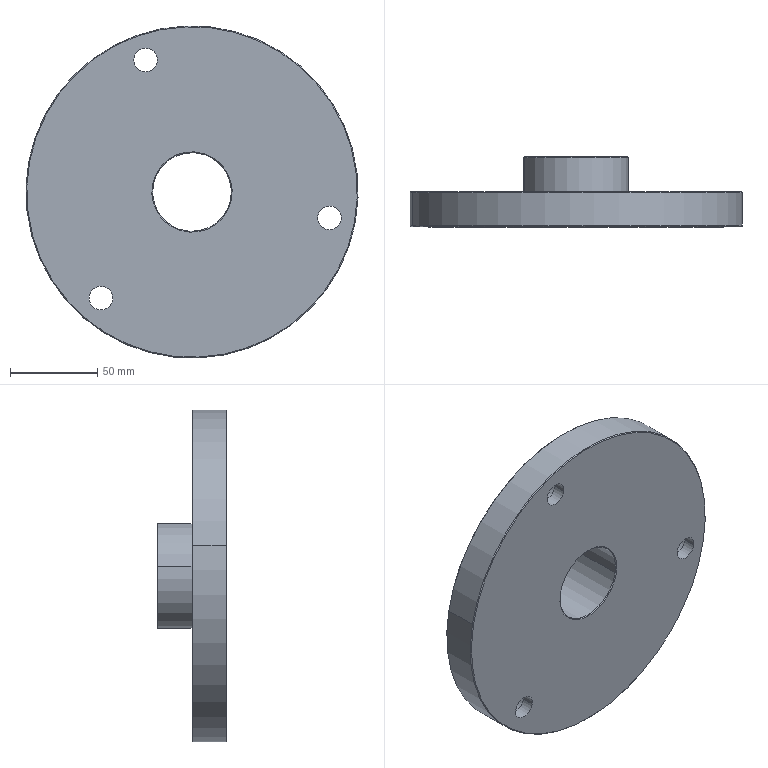Component | SolidWorks | 002AS-20130718-1_009A-20130717-1 | 1 solid | 34 faces | box 190 x 40 x 190 mm | volume 544523 mm3 | cylinder 18 | cone 10 | plane 6 | commonest cylinder face diameters 20 x6 13.5 x6 60 x2 45 x2 190 x2
STEP:
#1=COLOUR_RGB('',0.7922,0.8196,0.9333);
#2=FILL_AREA_STYLE_COLOUR('',#1);
#3=FILL_AREA_STYLE('',(#2));
#4=SURFACE_STYLE_FILL_AREA(#3);
#5=SURFACE_SIDE_STYLE('',(#4));
#6=SURFACE_STYLE_USAGE(.BOTH.,#5);
#7=PRESENTATION_STYLE_ASSIGNMENT((#6));
#8=CARTESIAN_POINT('',(-10.319,22.763,3.707));
#9=VERTEX_POINT('',#8);
#10=CARTESIAN_POINT('',(-8.578,22.763,3.38));
#11=VERTEX_POINT('',#10);
#12=CARTESIAN_POINT('',(-9.449,22.763,3.543));
#13=DIRECTION('',(-0.,-1.,0.));
#14=DIRECTION('',(-0.9828,0.,0.1846));
#15=AXIS2_PLACEMENT_3D('',#12,#13,#14);
#16=CIRCLE('',#15,0.8858);
#17=EDGE_CURVE('',#9,#11,#16,.T.);
#18=ORIENTED_EDGE('',*,*,#17,.F.);
#19=CARTESIAN_POINT('',(-10.339,22.743,3.71));
#20=VERTEX_POINT('',#19);
#21=CARTESIAN_POINT('',(-10.339,22.743,3.71));
#22=DIRECTION('',(-0.695,-0.7071,0.1305));
#23=VECTOR('',#22,39.37);
#24=LINE('',#21,#23);
#25=EDGE_CURVE('',#9,#20,#24,.T.);
#26=ORIENTED_EDGE('',*,*,#25,.T.);
#27=CARTESIAN_POINT('',(-8.559,22.743,3.376));
#28=VERTEX_POINT('',#27);
#29=CARTESIAN_POINT('',(-9.449,22.743,3.543));
#30=DIRECTION('',(0.,1.,-0.));
#31=DIRECTION('',(-0.9828,0.,0.1846));
#32=AXIS2_PLACEMENT_3D('',#29,#30,#31);
#33=CIRCLE('',#32,0.9055);
#34=EDGE_CURVE('',#28,#20,#33,.T.);
#35=ORIENTED_EDGE('',*,*,#34,.F.);
#36=CARTESIAN_POINT('',(-8.559,22.743,3.376));
#37=DIRECTION('',(0.695,-0.7071,-0.1305));
#38=VECTOR('',#37,39.37);
#39=LINE('',#36,#38);
#40=EDGE_CURVE('',#11,#28,#39,.T.);
#41=ORIENTED_EDGE('',*,*,#40,.F.);
#42=EDGE_LOOP('',(#18,#26,#35,#41));
#43=FACE_OUTER_BOUND('',#42,.T.);
#44=CARTESIAN_POINT('',(-9.449,22.743,3.543));
#45=DIRECTION('',(-0.,-1.,0.));
#46=DIRECTION('',(0.9828,0.,-0.1846));
#47=AXIS2_PLACEMENT_3D('',#44,#45,#46);
#48=CONICAL_SURFACE('',#47,0.9055,0.7854);
#49=ADVANCED_FACE('',(#43),#48,.F.);
#50=CARTESIAN_POINT('',(-10.59,24.318,3.758));
#51=VERTEX_POINT('',#50);
#52=CARTESIAN_POINT('',(-8.307,24.318,3.329));
#53=VERTEX_POINT('',#52);
#54=CARTESIAN_POINT('',(-9.449,24.318,3.543));
#55=DIRECTION('',(0.,1.,-0.));
#56=DIRECTION('',(-0.9828,0.,0.1846));
#57=AXIS2_PLACEMENT_3D('',#54,#55,#56);
#58=CIRCLE('',#57,1.161);
#59=EDGE_CURVE('',#51,#53,#58,.T.);
#60=ORIENTED_EDGE('',*,*,#59,.F.);
#61=CARTESIAN_POINT('',(-10.61,24.298,3.761));
#62=VERTEX_POINT('',#61);
#63=CARTESIAN_POINT('',(-10.59,24.318,3.758));
#64=DIRECTION('',(-0.695,-0.7071,0.1305));
#65=VECTOR('',#64,39.37);
#66=LINE('',#63,#65);
#67=EDGE_CURVE('',#51,#62,#66,.T.);
#68=ORIENTED_EDGE('',*,*,#67,.T.);
#69=CARTESIAN_POINT('',(-8.288,24.298,3.325));
#70=VERTEX_POINT('',#69);
#71=CARTESIAN_POINT('',(-9.449,24.298,3.543));
#72=DIRECTION('',(-0.,-1.,0.));
#73=DIRECTION('',(-0.9828,0.,0.1846));
#74=AXIS2_PLACEMENT_3D('',#71,#72,#73);
#75=CIRCLE('',#74,1.181);
#76=EDGE_CURVE('',#70,#62,#75,.T.);
#77=ORIENTED_EDGE('',*,*,#76,.F.);
#78=CARTESIAN_POINT('',(-8.307,24.318,3.329));
#79=DIRECTION('',(0.695,-0.7071,-0.1305));
#80=VECTOR('',#79,39.37);
#81=LINE('',#78,#80);
#82=EDGE_CURVE('',#53,#70,#81,.T.);
#83=ORIENTED_EDGE('',*,*,#82,.F.);
#84=EDGE_LOOP('',(#60,#68,#77,#83));
#85=FACE_OUTER_BOUND('',#84,.T.);
#86=CARTESIAN_POINT('',(-9.449,24.318,3.543));
#87=DIRECTION('',(-0.,-1.,0.));
#88=DIRECTION('',(0.9828,0.,-0.1846));
#89=AXIS2_PLACEMENT_3D('',#86,#87,#88);
#90=CONICAL_SURFACE('',#89,1.161,0.7854);
#91=ADVANCED_FACE('',(#85),#90,.T.);
#92=CARTESIAN_POINT('',(-8.578,24.298,3.38));
#93=VERTEX_POINT('',#92);
#94=CARTESIAN_POINT('',(-10.319,24.298,3.707));
#95=VERTEX_POINT('',#94);
#96=CARTESIAN_POINT('',(-9.449,24.298,3.543));
#97=DIRECTION('',(0.,1.,-0.));
#98=DIRECTION('',(-0.9828,0.,0.1846));
#99=AXIS2_PLACEMENT_3D('',#96,#97,#98);
#100=CIRCLE('',#99,0.8858);
#101=EDGE_CURVE('',#93,#95,#100,.T.);
#102=ORIENTED_EDGE('',*,*,#101,.F.);
#103=CARTESIAN_POINT('',(-8.559,24.318,3.376));
#104=VERTEX_POINT('',#103);
#105=CARTESIAN_POINT('',(-8.578,24.298,3.38));
#106=DIRECTION('',(0.695,0.7071,-0.1305));
#107=VECTOR('',#106,39.37);
#108=LINE('',#105,#107);
#109=EDGE_CURVE('',#93,#104,#108,.T.);
#110=ORIENTED_EDGE('',*,*,#109,.T.);
#111=CARTESIAN_POINT('',(-10.339,24.318,3.71));
#112=VERTEX_POINT('',#111);
#113=CARTESIAN_POINT('',(-9.449,24.318,3.543));
#114=DIRECTION('',(-0.,-1.,0.));
#115=DIRECTION('',(-0.9828,0.,0.1846));
#116=AXIS2_PLACEMENT_3D('',#113,#114,#115);
#117=CIRCLE('',#116,0.9055);
#118=EDGE_CURVE('',#112,#104,#117,.T.);
#119=ORIENTED_EDGE('',*,*,#118,.F.);
#120=CARTESIAN_POINT('',(-10.319,24.298,3.707));
#121=DIRECTION('',(-0.695,0.7071,0.1305));
#122=VECTOR('',#121,39.37);
#123=LINE('',#120,#122);
#124=EDGE_CURVE('',#95,#112,#123,.T.);
#125=ORIENTED_EDGE('',*,*,#124,.F.);
#126=EDGE_LOOP('',(#102,#110,#119,#125));
#127=FACE_OUTER_BOUND('',#126,.T.);
#128=CARTESIAN_POINT('',(-9.449,24.298,3.543));
#129=DIRECTION('',(0.,1.,-0.));
#130=DIRECTION('',(-0.9828,0.,0.1846));
#131=AXIS2_PLACEMENT_3D('',#128,#129,#130);
#132=CONICAL_SURFACE('',#131,0.8858,0.7854);
#133=ADVANCED_FACE('',(#127),#132,.F.);
#134=CARTESIAN_POINT('',(-11.113,23.019,1.081));
#135=VERTEX_POINT('',#134);
#136=CARTESIAN_POINT('',(-11.887,23.019,1.226));
#137=VERTEX_POINT('',#136);
#138=CARTESIAN_POINT('',(-11.5,23.019,1.153));
#139=DIRECTION('',(0.,1.,-0.));
#140=DIRECTION('',(-0.9828,0.,0.1846));
#141=AXIS2_PLACEMENT_3D('',#138,#139,#140);
#142=CIRCLE('',#141,0.3937);
#143=EDGE_CURVE('',#135,#137,#142,.T.);
#144=ORIENTED_EDGE('',*,*,#143,.F.);
#145=CARTESIAN_POINT('',(-11.113,23.531,1.081));
#146=VERTEX_POINT('',#145);
#147=CARTESIAN_POINT('',(-11.113,23.531,1.081));
#148=DIRECTION('',(0.,1.,-0.));
#149=VECTOR('',#148,39.37);
#150=LINE('',#147,#149);
#151=EDGE_CURVE('',#135,#146,#150,.T.);
#152=ORIENTED_EDGE('',*,*,#151,.T.);
#153=CARTESIAN_POINT('',(-11.887,23.531,1.226));
#154=VERTEX_POINT('',#153);
#155=CARTESIAN_POINT('',(-11.5,23.531,1.153));
#156=DIRECTION('',(0.,1.,-0.));
#157=DIRECTION('',(-0.9828,0.,0.1846));
#158=AXIS2_PLACEMENT_3D('',#155,#156,#157);
#159=CIRCLE('',#158,0.3937);
#160=EDGE_CURVE('',#146,#154,#159,.T.);
#161=ORIENTED_EDGE('',*,*,#160,.T.);
#162=CARTESIAN_POINT('',(-11.887,23.531,1.226));
#163=DIRECTION('',(0.,1.,-0.));
#164=VECTOR('',#163,39.37);
#165=LINE('',#162,#164);
#166=EDGE_CURVE('',#137,#154,#165,.T.);
#167=ORIENTED_EDGE('',*,*,#166,.F.);
#168=EDGE_LOOP('',(#144,#152,#161,#167));
#169=FACE_OUTER_BOUND('',#168,.T.);
#170=CARTESIAN_POINT('',(-11.5,23.531,1.153));
#171=DIRECTION('',(0.,1.,-0.));
#172=DIRECTION('',(-0.9828,0.,0.1846));
#173=AXIS2_PLACEMENT_3D('',#170,#171,#172);
#174=CYLINDRICAL_SURFACE('',#173,0.3937);
#175=ADVANCED_FACE('',(#169),#174,.F.);
#176=CARTESIAN_POINT('',(-11.239,22.743,1.104));
#177=VERTEX_POINT('',#176);
#178=CARTESIAN_POINT('',(-11.761,22.743,1.202));
#179=VERTEX_POINT('',#178);
#180=CARTESIAN_POINT('',(-11.5,22.743,1.153));
#181=DIRECTION('',(0.,1.,-0.));
#182=DIRECTION('',(-0.9828,0.,0.1846));
#183=AXIS2_PLACEMENT_3D('',#180,#181,#182);
#184=CIRCLE('',#183,0.2657);
#185=EDGE_CURVE('',#177,#179,#184,.T.);
#186=ORIENTED_EDGE('',*,*,#185,.F.);
#187=CARTESIAN_POINT('',(-11.239,23.019,1.104));
#188=VERTEX_POINT('',#187);
#189=CARTESIAN_POINT('',(-11.239,23.531,1.104));
#190=DIRECTION('',(0.,1.,-0.));
#191=VECTOR('',#190,39.37);
#192=LINE('',#189,#191);
#193=EDGE_CURVE('',#177,#188,#192,.T.);
#194=ORIENTED_EDGE('',*,*,#193,.T.);
#195=CARTESIAN_POINT('',(-11.761,23.019,1.202));
#196=VERTEX_POINT('',#195);
#197=CARTESIAN_POINT('',(-11.5,23.019,1.153));
#198=DIRECTION('',(0.,1.,-0.));
#199=DIRECTION('',(-0.9828,0.,0.1846));
#200=AXIS2_PLACEMENT_3D('',#197,#198,#199);
#201=CIRCLE('',#200,0.2657);
#202=EDGE_CURVE('',#188,#196,#201,.T.);
#203=ORIENTED_EDGE('',*,*,#202,.T.);
#204=CARTESIAN_POINT('',(-11.761,23.531,1.202));
#205=DIRECTION('',(0.,1.,-0.));
#206=VECTOR('',#205,39.37);
#207=LINE('',#204,#206);
#208=EDGE_CURVE('',#179,#196,#207,.T.);
#209=ORIENTED_EDGE('',*,*,#208,.F.);
#210=EDGE_LOOP('',(#186,#194,#203,#209));
#211=FACE_OUTER_BOUND('',#210,.T.);
#212=CARTESIAN_POINT('',(-11.5,23.531,1.153));
#213=DIRECTION('',(0.,1.,-0.));
#214=DIRECTION('',(-0.9828,0.,0.1846));
#215=AXIS2_PLACEMENT_3D('',#212,#213,#214);
#216=CYLINDRICAL_SURFACE('',#215,0.2657);
#217=ADVANCED_FACE('',(#211),#216,.F.);
#218=CARTESIAN_POINT('',(-10.106,23.019,6.442));
#219=VERTEX_POINT('',#218);
#220=CARTESIAN_POINT('',(-10.88,23.019,6.587));
#221=VERTEX_POINT('',#220);
#222=CARTESIAN_POINT('',(-10.493,23.019,6.515));
#223=DIRECTION('',(0.,1.,-0.));
#224=DIRECTION('',(-0.9828,0.,0.1846));
#225=AXIS2_PLACEMENT_3D('',#222,#223,#224);
#226=CIRCLE('',#225,0.3937);
#227=EDGE_CURVE('',#219,#221,#226,.T.);
#228=ORIENTED_EDGE('',*,*,#227,.F.);
#229=CARTESIAN_POINT('',(-10.106,23.531,6.442));
#230=VERTEX_POINT('',#229);
#231=CARTESIAN_POINT('',(-10.106,23.531,6.442));
#232=DIRECTION('',(0.,1.,-0.));
#233=VECTOR('',#232,39.37);
#234=LINE('',#231,#233);
#235=EDGE_CURVE('',#219,#230,#234,.T.);
#236=ORIENTED_EDGE('',*,*,#235,.T.);
#237=CARTESIAN_POINT('',(-10.88,23.531,6.587));
#238=VERTEX_POINT('',#237);
#239=CARTESIAN_POINT('',(-10.493,23.531,6.515));
#240=DIRECTION('',(0.,1.,-0.));
#241=DIRECTION('',(-0.9828,0.,0.1846));
#242=AXIS2_PLACEMENT_3D('',#239,#240,#241);
#243=CIRCLE('',#242,0.3937);
#244=EDGE_CURVE('',#230,#238,#243,.T.);
#245=ORIENTED_EDGE('',*,*,#244,.T.);
#246=CARTESIAN_POINT('',(-10.88,23.531,6.587));
#247=DIRECTION('',(0.,1.,-0.));
#248=VECTOR('',#247,39.37);
#249=LINE('',#246,#248);
#250=EDGE_CURVE('',#221,#238,#249,.T.);
#251=ORIENTED_EDGE('',*,*,#250,.F.);
#252=EDGE_LOOP('',(#228,#236,#245,#251));
#253=FACE_OUTER_BOUND('',#252,.T.);
#254=CARTESIAN_POINT('',(-10.493,23.531,6.515));
#255=DIRECTION('',(0.,1.,-0.));
#256=DIRECTION('',(-0.9828,0.,0.1846));
#257=AXIS2_PLACEMENT_3D('',#254,#255,#256);
#258=CYLINDRICAL_SURFACE('',#257,0.3937);
#259=ADVANCED_FACE('',(#253),#258,.F.);
#260=CARTESIAN_POINT('',(-10.232,22.743,6.466));
#261=VERTEX_POINT('',#260);
#262=CARTESIAN_POINT('',(-10.754,22.743,6.564));
#263=VERTEX_POINT('',#262);
#264=CARTESIAN_POINT('',(-10.493,22.743,6.515));
#265=DIRECTION('',(0.,1.,-0.));
#266=DIRECTION('',(-0.9828,0.,0.1846));
#267=AXIS2_PLACEMENT_3D('',#264,#265,#266);
#268=CIRCLE('',#267,0.2657);
#269=EDGE_CURVE('',#261,#263,#268,.T.);
#270=ORIENTED_EDGE('',*,*,#269,.F.);
#271=CARTESIAN_POINT('',(-10.232,23.019,6.466));
#272=VERTEX_POINT('',#271);
#273=CARTESIAN_POINT('',(-10.232,23.531,6.466));
#274=DIRECTION('',(0.,1.,-0.));
#275=VECTOR('',#274,39.37);
#276=LINE('',#273,#275);
#277=EDGE_CURVE('',#261,#272,#276,.T.);
#278=ORIENTED_EDGE('',*,*,#277,.T.);
#279=CARTESIAN_POINT('',(-10.754,23.019,6.564));
#280=VERTEX_POINT('',#279);
#281=CARTESIAN_POINT('',(-10.493,23.019,6.515));
#282=DIRECTION('',(0.,1.,-0.));
#283=DIRECTION('',(-0.9828,0.,0.1846));
#284=AXIS2_PLACEMENT_3D('',#281,#282,#283);
#285=CIRCLE('',#284,0.2657);
#286=EDGE_CURVE('',#272,#280,#285,.T.);
#287=ORIENTED_EDGE('',*,*,#286,.T.);
#288=CARTESIAN_POINT('',(-10.754,23.531,6.564));
#289=DIRECTION('',(0.,1.,-0.));
#290=VECTOR('',#289,39.37);
#291=LINE('',#288,#290);
#292=EDGE_CURVE('',#263,#280,#291,.T.);
#293=ORIENTED_EDGE('',*,*,#292,.F.);
#294=EDGE_LOOP('',(#270,#278,#287,#293));
#295=FACE_OUTER_BOUND('',#294,.T.);
#296=CARTESIAN_POINT('',(-10.493,23.531,6.515));
#297=DIRECTION('',(0.,1.,-0.));
#298=DIRECTION('',(-0.9828,0.,0.1846));
#299=AXIS2_PLACEMENT_3D('',#296,#297,#298);
#300=CYLINDRICAL_SURFACE('',#299,0.2657);
#301=ADVANCED_FACE('',(#295),#300,.F.);
#302=CARTESIAN_POINT('',(-13.105,23.531,4.23));
#303=VERTEX_POINT('',#302);
#304=CARTESIAN_POINT('',(-5.792,23.531,2.857));
#305=VERTEX_POINT('',#304);
#306=CARTESIAN_POINT('',(-9.449,23.531,3.543));
#307=DIRECTION('',(0.,1.,-0.));
#308=DIRECTION('',(-0.9828,0.,0.1846));
#309=AXIS2_PLACEMENT_3D('',#306,#307,#308);
#310=CIRCLE('',#309,3.72);
#311=EDGE_CURVE('',#303,#305,#310,.T.);
#312=ORIENTED_EDGE('',*,*,#311,.F.);
#313=CARTESIAN_POINT('',(-13.125,23.511,4.234));
#314=VERTEX_POINT('',#313);
#315=CARTESIAN_POINT('',(-13.105,23.531,4.23));
#316=DIRECTION('',(-0.695,-0.7071,0.1305));
#317=VECTOR('',#316,39.37);
#318=LINE('',#315,#317);
#319=EDGE_CURVE('',#303,#314,#318,.T.);
#320=ORIENTED_EDGE('',*,*,#319,.T.);
#321=CARTESIAN_POINT('',(-5.773,23.511,2.853));
#322=VERTEX_POINT('',#321);
#323=CARTESIAN_POINT('',(-9.449,23.511,3.543));
#324=DIRECTION('',(-0.,-1.,0.));
#325=DIRECTION('',(-0.9828,0.,0.1846));
#326=AXIS2_PLACEMENT_3D('',#323,#324,#325);
#327=CIRCLE('',#326,3.74);
#328=EDGE_CURVE('',#322,#314,#327,.T.);
#329=ORIENTED_EDGE('',*,*,#328,.F.);
#330=CARTESIAN_POINT('',(-5.792,23.531,2.857));
#331=DIRECTION('',(0.695,-0.7071,-0.1305));
#332=VECTOR('',#331,39.37);
#333=LINE('',#330,#332);
#334=EDGE_CURVE('',#305,#322,#333,.T.);
#335=ORIENTED_EDGE('',*,*,#334,.F.);
#336=EDGE_LOOP('',(#312,#320,#329,#335));
#337=FACE_OUTER_BOUND('',#336,.T.);
#338=CARTESIAN_POINT('',(-9.449,23.531,3.543));
#339=DIRECTION('',(-0.,-1.,0.));
#340=DIRECTION('',(0.9828,0.,-0.1846));
#341=AXIS2_PLACEMENT_3D('',#338,#339,#340);
#342=CONICAL_SURFACE('',#341,3.72,0.7854);
#343=ADVANCED_FACE('',(#337),#342,.T.);
#344=CARTESIAN_POINT('',(-5.792,22.743,2.857));
#345=VERTEX_POINT('',#344);
#346=CARTESIAN_POINT('',(-13.105,22.743,4.23));
#347=VERTEX_POINT('',#346);
#348=CARTESIAN_POINT('',(-9.449,22.743,3.543));
#349=DIRECTION('',(-0.,-1.,0.));
#350=DIRECTION('',(-0.9828,0.,0.1846));
#351=AXIS2_PLACEMENT_3D('',#348,#349,#350);
#352=CIRCLE('',#351,3.72);
#353=EDGE_CURVE('',#345,#347,#352,.T.);
#354=ORIENTED_EDGE('',*,*,#353,.F.);
#355=CARTESIAN_POINT('',(-5.773,22.763,2.853));
#356=VERTEX_POINT('',#355);
#357=CARTESIAN_POINT('',(-5.773,22.763,2.853));
#358=DIRECTION('',(0.695,0.7071,-0.1305));
#359=VECTOR('',#358,39.37);
#360=LINE('',#357,#359);
#361=EDGE_CURVE('',#345,#356,#360,.T.);
#362=ORIENTED_EDGE('',*,*,#361,.T.);
#363=CARTESIAN_POINT('',(-13.125,22.763,4.234));
#364=VERTEX_POINT('',#363);
#365=CARTESIAN_POINT('',(-9.449,22.763,3.543));
#366=DIRECTION('',(0.,1.,-0.));
#367=DIRECTION('',(-0.9828,0.,0.1846));
#368=AXIS2_PLACEMENT_3D('',#365,#366,#367);
#369=CIRCLE('',#368,3.74);
#370=EDGE_CURVE('',#364,#356,#369,.T.);
#371=ORIENTED_EDGE('',*,*,#370,.F.);
#372=CARTESIAN_POINT('',(-13.125,22.763,4.234));
#373=DIRECTION('',(-0.695,0.7071,0.1305));
#374=VECTOR('',#373,39.37);
#375=LINE('',#372,#374);
#376=EDGE_CURVE('',#347,#364,#375,.T.);
#377=ORIENTED_EDGE('',*,*,#376,.F.);
#378=EDGE_LOOP('',(#354,#362,#371,#377));
#379=FACE_OUTER_BOUND('',#378,.T.);
#380=CARTESIAN_POINT('',(-9.449,22.763,3.543));
#381=DIRECTION('',(0.,1.,-0.));
#382=DIRECTION('',(-0.9828,0.,0.1846));
#383=AXIS2_PLACEMENT_3D('',#380,#381,#382);
#384=CONICAL_SURFACE('',#383,3.74,0.7854);
#385=ADVANCED_FACE('',(#379),#384,.T.);
#386=CARTESIAN_POINT('',(-5.966,23.019,2.889));
#387=VERTEX_POINT('',#386);
#388=CARTESIAN_POINT('',(-6.74,23.019,3.035));
#389=VERTEX_POINT('',#388);
#390=CARTESIAN_POINT('',(-6.353,23.019,2.962));
#391=DIRECTION('',(0.,1.,-0.));
#392=DIRECTION('',(-0.9828,0.,0.1846));
#393=AXIS2_PLACEMENT_3D('',#390,#391,#392);
#394=CIRCLE('',#393,0.3937);
#395=EDGE_CURVE('',#387,#389,#394,.T.);
#396=ORIENTED_EDGE('',*,*,#395,.F.);
#397=CARTESIAN_POINT('',(-5.966,23.531,2.889));
#398=VERTEX_POINT('',#397);
#399=CARTESIAN_POINT('',(-5.966,23.531,2.889));
#400=DIRECTION('',(0.,1.,-0.));
#401=VECTOR('',#400,39.37);
#402=LINE('',#399,#401);
#403=EDGE_CURVE('',#387,#398,#402,.T.);
#404=ORIENTED_EDGE('',*,*,#403,.T.);
#405=CARTESIAN_POINT('',(-6.74,23.531,3.035));
#406=VERTEX_POINT('',#405);
#407=CARTESIAN_POINT('',(-6.353,23.531,2.962));
#408=DIRECTION('',(0.,1.,-0.));
#409=DIRECTION('',(-0.9828,0.,0.1846));
#410=AXIS2_PLACEMENT_3D('',#407,#408,#409);
#411=CIRCLE('',#410,0.3937);
#412=EDGE_CURVE('',#398,#406,#411,.T.);
#413=ORIENTED_EDGE('',*,*,#412,.T.);
#414=CARTESIAN_POINT('',(-6.74,23.531,3.035));
#415=DIRECTION('',(0.,1.,-0.));
#416=VECTOR('',#415,39.37);
#417=LINE('',#414,#416);
#418=EDGE_CURVE('',#389,#406,#417,.T.);
#419=ORIENTED_EDGE('',*,*,#418,.F.);
#420=EDGE_LOOP('',(#396,#404,#413,#419));
#421=FACE_OUTER_BOUND('',#420,.T.);
#422=CARTESIAN_POINT('',(-6.353,23.531,2.962));
#423=DIRECTION('',(0.,1.,-0.));
#424=DIRECTION('',(-0.9828,0.,0.1846));
#425=AXIS2_PLACEMENT_3D('',#422,#423,#424);
#426=CYLINDRICAL_SURFACE('',#425,0.3937);
#427=ADVANCED_FACE('',(#421),#426,.F.);
#428=CARTESIAN_POINT('',(-6.092,22.743,2.913));
#429=VERTEX_POINT('',#428);
#430=CARTESIAN_POINT('',(-6.615,22.743,3.011));
#431=VERTEX_POINT('',#430);
#432=CARTESIAN_POINT('',(-6.353,22.743,2.962));
#433=DIRECTION('',(0.,1.,-0.));
#434=DIRECTION('',(-0.9828,0.,0.1846));
#435=AXIS2_PLACEMENT_3D('',#432,#433,#434);
#436=CIRCLE('',#435,0.2657);
#437=EDGE_CURVE('',#429,#431,#436,.T.);
#438=ORIENTED_EDGE('',*,*,#437,.F.);
#439=CARTESIAN_POINT('',(-6.092,23.019,2.913));
#440=VERTEX_POINT('',#439);
#441=CARTESIAN_POINT('',(-6.092,23.531,2.913));
#442=DIRECTION('',(0.,1.,-0.));
#443=VECTOR('',#442,39.37);
#444=LINE('',#441,#443);
#445=EDGE_CURVE('',#429,#440,#444,.T.);
#446=ORIENTED_EDGE('',*,*,#445,.T.);
#447=CARTESIAN_POINT('',(-6.615,23.019,3.011));
#448=VERTEX_POINT('',#447);
#449=CARTESIAN_POINT('',(-6.353,23.019,2.962));
#450=DIRECTION('',(0.,1.,-0.));
#451=DIRECTION('',(-0.9828,0.,0.1846));
#452=AXIS2_PLACEMENT_3D('',#449,#450,#451);
#453=CIRCLE('',#452,0.2657);
#454=EDGE_CURVE('',#440,#448,#453,.T.);
#455=ORIENTED_EDGE('',*,*,#454,.T.);
#456=CARTESIAN_POINT('',(-6.615,23.531,3.011));
#457=DIRECTION('',(0.,1.,-0.));
#458=VECTOR('',#457,39.37);
#459=LINE('',#456,#458);
#460=EDGE_CURVE('',#431,#448,#459,.T.);
#461=ORIENTED_EDGE('',*,*,#460,.F.);
#462=EDGE_LOOP('',(#438,#446,#455,#461));
#463=FACE_OUTER_BOUND('',#462,.T.);
#464=CARTESIAN_POINT('',(-6.353,23.531,2.962));
#465=DIRECTION('',(0.,1.,-0.));
#466=DIRECTION('',(-0.9828,0.,0.1846));
#467=AXIS2_PLACEMENT_3D('',#464,#465,#466);
#468=CYLINDRICAL_SURFACE('',#467,0.2657);
#469=ADVANCED_FACE('',(#463),#468,.F.);
#470=ORIENTED_EDGE('',*,*,#76,.T.);
#471=CARTESIAN_POINT('',(-10.61,23.531,3.761));
#472=VERTEX_POINT('',#471);
#473=CARTESIAN_POINT('',(-10.61,24.318,3.761));
#474=DIRECTION('',(-0.,-1.,0.));
#475=VECTOR('',#474,39.37);
#476=LINE('',#473,#475);
#477=EDGE_CURVE('',#62,#472,#476,.T.);
#478=ORIENTED_EDGE('',*,*,#477,.T.);
#479=CARTESIAN_POINT('',(-8.288,23.531,3.325));
#480=VERTEX_POINT('',#479);
#481=CARTESIAN_POINT('',(-9.449,23.531,3.543));
#482=DIRECTION('',(0.,1.,-0.));
#483=DIRECTION('',(-0.9828,0.,0.1846));
#484=AXIS2_PLACEMENT_3D('',#481,#482,#483);
#485=CIRCLE('',#484,1.181);
#486=EDGE_CURVE('',#472,#480,#485,.T.);
#487=ORIENTED_EDGE('',*,*,#486,.T.);
#488=CARTESIAN_POINT('',(-8.288,24.318,3.325));
#489=DIRECTION('',(-0.,-1.,0.));
#490=VECTOR('',#489,39.37);
#491=LINE('',#488,#490);
#492=EDGE_CURVE('',#70,#480,#491,.T.);
#493=ORIENTED_EDGE('',*,*,#492,.F.);
#494=EDGE_LOOP('',(#470,#478,#487,#493));
#495=FACE_OUTER_BOUND('',#494,.T.);
#496=CARTESIAN_POINT('',(-9.449,24.318,3.543));
#497=DIRECTION('',(-0.,-1.,0.));
#498=DIRECTION('',(0.9828,0.,-0.1846));
#499=AXIS2_PLACEMENT_3D('',#496,#497,#498);
#500=CYLINDRICAL_SURFACE('',#499,1.181);
#501=ADVANCED_FACE('',(#495),#500,.T.);
#502=ORIENTED_EDGE('',*,*,#101,.T.);
#503=CARTESIAN_POINT('',(-10.319,23.531,3.707));
#504=DIRECTION('',(-0.,-1.,0.));
#505=VECTOR('',#504,39.37);
#506=LINE('',#503,#505);
#507=EDGE_CURVE('',#95,#9,#506,.T.);
#508=ORIENTED_EDGE('',*,*,#507,.T.);
#509=ORIENTED_EDGE('',*,*,#17,.T.);
#510=CARTESIAN_POINT('',(-8.578,23.531,3.38));
#511=DIRECTION('',(-0.,-1.,0.));
#512=VECTOR('',#511,39.37);
#513=LINE('',#510,#512);
#514=EDGE_CURVE('',#93,#11,#513,.T.);
#515=ORIENTED_EDGE('',*,*,#514,.F.);
#516=EDGE_LOOP('',(#502,#508,#509,#515));
#517=FACE_OUTER_BOUND('',#516,.T.);
#518=CARTESIAN_POINT('',(-9.449,23.531,3.543));
#519=DIRECTION('',(-0.,-1.,0.));
#520=DIRECTION('',(0.9828,0.,-0.1846));
#521=AXIS2_PLACEMENT_3D('',#518,#519,#520);
#522=CYLINDRICAL_SURFACE('',#521,0.8858);
#523=ADVANCED_FACE('',(#517),#522,.F.);
#524=ORIENTED_EDGE('',*,*,#328,.T.);
#525=CARTESIAN_POINT('',(-13.125,23.531,4.234));
#526=DIRECTION('',(-0.,-1.,0.));
#527=VECTOR('',#526,39.37);
#528=LINE('',#525,#527);
#529=EDGE_CURVE('',#314,#364,#528,.T.);
#530=ORIENTED_EDGE('',*,*,#529,.T.);
#531=ORIENTED_EDGE('',*,*,#370,.T.);
#532=CARTESIAN_POINT('',(-5.773,23.531,2.853));
#533=DIRECTION('',(-0.,-1.,0.));
#534=VECTOR('',#533,39.37);
#535=LINE('',#532,#534);
#536=EDGE_CURVE('',#322,#356,#535,.T.);
#537=ORIENTED_EDGE('',*,*,#536,.F.);
#538=EDGE_LOOP('',(#524,#530,#531,#537));
#539=FACE_OUTER_BOUND('',#538,.T.);
#540=CARTESIAN_POINT('',(-9.449,23.531,3.543));
#541=DIRECTION('',(-0.,-1.,0.));
#542=DIRECTION('',(0.9828,0.,-0.1846));
#543=AXIS2_PLACEMENT_3D('',#540,#541,#542);
#544=CYLINDRICAL_SURFACE('',#543,3.74);
#545=ADVANCED_FACE('',(#539),#544,.T.);
#546=CARTESIAN_POINT('',(-11.5,23.531,1.153));
#547=DIRECTION('',(0.,1.,-0.));
#548=DIRECTION('',(-0.9828,0.,0.1846));
#549=AXIS2_PLACEMENT_3D('',#546,#547,#548);
#550=CIRCLE('',#549,0.3937);
#551=EDGE_CURVE('',#154,#146,#550,.T.);
#552=ORIENTED_EDGE('',*,*,#551,.F.);
#553=ORIENTED_EDGE('',*,*,#160,.F.);
#554=EDGE_LOOP('',(#552,#553));
#555=FACE_BOUND('',#554,.T.);
#556=CARTESIAN_POINT('',(-10.493,23.531,6.515));
#557=DIRECTION('',(0.,1.,-0.));
#558=DIRECTION('',(-0.9828,0.,0.1846));
#559=AXIS2_PLACEMENT_3D('',#556,#557,#558);
#560=CIRCLE('',#559,0.3937);
#561=EDGE_CURVE('',#238,#230,#560,.T.);
#562=ORIENTED_EDGE('',*,*,#561,.F.);
#563=ORIENTED_EDGE('',*,*,#244,.F.);
#564=EDGE_LOOP('',(#562,#563));
#565=FACE_BOUND('',#564,.T.);
#566=CARTESIAN_POINT('',(-9.449,23.531,3.543));
#567=DIRECTION('',(0.,1.,-0.));
#568=DIRECTION('',(-0.9828,0.,0.1846));
#569=AXIS2_PLACEMENT_3D('',#566,#567,#568);
#570=CIRCLE('',#569,3.72);
#571=EDGE_CURVE('',#305,#303,#570,.T.);
#572=ORIENTED_EDGE('',*,*,#571,.T.);
#573=ORIENTED_EDGE('',*,*,#311,.T.);
#574=EDGE_LOOP('',(#572,#573));
#575=FACE_OUTER_BOUND('',#574,.T.);
#576=CARTESIAN_POINT('',(-6.353,23.531,2.962));
#577=DIRECTION('',(0.,1.,-0.));
#578=DIRECTION('',(-0.9828,0.,0.1846));
#579=AXIS2_PLACEMENT_3D('',#576,#577,#578);
#580=CIRCLE('',#579,0.3937);
#581=EDGE_CURVE('',#406,#398,#580,.T.);
#582=ORIENTED_EDGE('',*,*,#581,.F.);
#583=ORIENTED_EDGE('',*,*,#412,.F.);
#584=EDGE_LOOP('',(#582,#583));
#585=FACE_BOUND('',#584,.T.);
#586=CARTESIAN_POINT('',(-9.449,23.531,3.543));
#587=DIRECTION('',(0.,1.,-0.));
#588=DIRECTION('',(-0.9828,0.,0.1846));
#589=AXIS2_PLACEMENT_3D('',#586,#587,#588);
#590=CIRCLE('',#589,1.181);
#591=EDGE_CURVE('',#480,#472,#590,.T.);
#592=ORIENTED_EDGE('',*,*,#591,.F.);
#593=ORIENTED_EDGE('',*,*,#486,.F.);
#594=EDGE_LOOP('',(#592,#593));
#595=FACE_BOUND('',#594,.T.);
#596=CARTESIAN_POINT('',(-9.449,23.531,3.543));
#597=DIRECTION('',(0.,1.,-0.));
#598=DIRECTION('',(-0.9828,0.,0.1846));
#599=AXIS2_PLACEMENT_3D('',#596,#597,#598);
#600=PLANE('',#599);
#601=ADVANCED_FACE('',(#555,#565,#575,#585,#595),#600,.T.);
#602=ORIENTED_EDGE('',*,*,#34,.T.);
#603=CARTESIAN_POINT('',(-9.449,22.743,3.543));
#604=DIRECTION('',(0.,1.,-0.));
#605=DIRECTION('',(-0.9828,0.,0.1846));
#606=AXIS2_PLACEMENT_3D('',#603,#604,#605);
#607=CIRCLE('',#606,0.9055);
#608=EDGE_CURVE('',#20,#28,#607,.T.);
#609=ORIENTED_EDGE('',*,*,#608,.T.);
#610=EDGE_LOOP('',(#602,#609));
#611=FACE_BOUND('',#610,.T.);
#612=CARTESIAN_POINT('',(-11.5,22.743,1.153));
#613=DIRECTION('',(0.,1.,-0.));
#614=DIRECTION('',(-0.9828,0.,0.1846));
#615=AXIS2_PLACEMENT_3D('',#612,#613,#614);
#616=CIRCLE('',#615,0.2657);
#617=EDGE_CURVE('',#179,#177,#616,.T.);
#618=ORIENTED_EDGE('',*,*,#617,.T.);
#619=ORIENTED_EDGE('',*,*,#185,.T.);
#620=EDGE_LOOP('',(#618,#619));
#621=FACE_BOUND('',#620,.T.);
#622=CARTESIAN_POINT('',(-10.493,22.743,6.515));
#623=DIRECTION('',(0.,1.,-0.));
#624=DIRECTION('',(-0.9828,0.,0.1846));
#625=AXIS2_PLACEMENT_3D('',#622,#623,#624);
#626=CIRCLE('',#625,0.2657);
#627=EDGE_CURVE('',#263,#261,#626,.T.);
#628=ORIENTED_EDGE('',*,*,#627,.T.);
#629=ORIENTED_EDGE('',*,*,#269,.T.);
#630=EDGE_LOOP('',(#628,#629));
#631=FACE_BOUND('',#630,.T.);
#632=CARTESIAN_POINT('',(-9.449,22.743,3.543));
#633=DIRECTION('',(-0.,-1.,0.));
#634=DIRECTION('',(-0.9828,0.,0.1846));
#635=AXIS2_PLACEMENT_3D('',#632,#633,#634);
#636=CIRCLE('',#635,3.72);
#637=EDGE_CURVE('',#347,#345,#636,.T.);
#638=ORIENTED_EDGE('',*,*,#637,.T.);
#639=ORIENTED_EDGE('',*,*,#353,.T.);
#640=EDGE_LOOP('',(#638,#639));
#641=FACE_OUTER_BOUND('',#640,.T.);
#642=CARTESIAN_POINT('',(-6.353,22.743,2.962));
#643=DIRECTION('',(0.,1.,-0.));
#644=DIRECTION('',(-0.9828,0.,0.1846));
#645=AXIS2_PLACEMENT_3D('',#642,#643,#644);
#646=CIRCLE('',#645,0.2657);
#647=EDGE_CURVE('',#431,#429,#646,.T.);
#648=ORIENTED_EDGE('',*,*,#647,.T.);
#649=ORIENTED_EDGE('',*,*,#437,.T.);
#650=EDGE_LOOP('',(#648,#649));
#651=FACE_BOUND('',#650,.T.);
#652=CARTESIAN_POINT('',(-9.449,22.743,3.543));
#653=DIRECTION('',(0.,1.,-0.));
#654=DIRECTION('',(-0.9828,0.,0.1846));
#655=AXIS2_PLACEMENT_3D('',#652,#653,#654);
#656=PLANE('',#655);
#657=ADVANCED_FACE('',(#611,#621,#631,#641,#651),#656,.F.);
#658=ORIENTED_EDGE('',*,*,#529,.F.);
#659=CARTESIAN_POINT('',(-9.449,23.511,3.543));
#660=DIRECTION('',(-0.,-1.,0.));
#661=DIRECTION('',(-0.9828,0.,0.1846));
#662=AXIS2_PLACEMENT_3D('',#659,#660,#661);
#663=CIRCLE('',#662,3.74);
#664=EDGE_CURVE('',#314,#322,#663,.T.);
#665=ORIENTED_EDGE('',*,*,#664,.T.);
#666=ORIENTED_EDGE('',*,*,#536,.T.);
#667=CARTESIAN_POINT('',(-9.449,22.763,3.543));
#668=DIRECTION('',(0.,1.,-0.));
#669=DIRECTION('',(-0.9828,0.,0.1846));
#670=AXIS2_PLACEMENT_3D('',#667,#668,#669);
#671=CIRCLE('',#670,3.74);
#672=EDGE_CURVE('',#356,#364,#671,.T.);
#673=ORIENTED_EDGE('',*,*,#672,.T.);
#674=EDGE_LOOP('',(#658,#665,#666,#673));
#675=FACE_OUTER_BOUND('',#674,.T.);
#676=CARTESIAN_POINT('',(-9.449,23.531,3.543));
#677=DIRECTION('',(-0.,-1.,0.));
#678=DIRECTION('',(0.9828,0.,-0.1846));
#679=AXIS2_PLACEMENT_3D('',#676,#677,#678);
#680=CYLINDRICAL_SURFACE('',#679,3.74);
#681=ADVANCED_FACE('',(#675),#680,.T.);
#682=ORIENTED_EDGE('',*,*,#507,.F.);
#683=CARTESIAN_POINT('',(-9.449,24.298,3.543));
#684=DIRECTION('',(0.,1.,-0.));
#685=DIRECTION('',(-0.9828,0.,0.1846));
#686=AXIS2_PLACEMENT_3D('',#683,#684,#685);
#687=CIRCLE('',#686,0.8858);
#688=EDGE_CURVE('',#95,#93,#687,.T.);
#689=ORIENTED_EDGE('',*,*,#688,.T.);
#690=ORIENTED_EDGE('',*,*,#514,.T.);
#691=CARTESIAN_POINT('',(-9.449,22.763,3.543));
#692=DIRECTION('',(-0.,-1.,0.));
#693=DIRECTION('',(-0.9828,0.,0.1846));
#694=AXIS2_PLACEMENT_3D('',#691,#692,#693);
#695=CIRCLE('',#694,0.8858);
#696=EDGE_CURVE('',#11,#9,#695,.T.);
#697=ORIENTED_EDGE('',*,*,#696,.T.);
#698=EDGE_LOOP('',(#682,#689,#690,#697));
#699=FACE_OUTER_BOUND('',#698,.T.);
#700=CARTESIAN_POINT('',(-9.449,23.531,3.543));
#701=DIRECTION('',(-0.,-1.,0.));
#702=DIRECTION('',(0.9828,0.,-0.1846));
#703=AXIS2_PLACEMENT_3D('',#700,#701,#702);
#704=CYLINDRICAL_SURFACE('',#703,0.8858);
#705=ADVANCED_FACE('',(#699),#704,.F.);
#706=ORIENTED_EDGE('',*,*,#118,.T.);
#707=CARTESIAN_POINT('',(-9.449,24.318,3.543));
#708=DIRECTION('',(-0.,-1.,0.));
#709=DIRECTION('',(-0.9828,0.,0.1846));
#710=AXIS2_PLACEMENT_3D('',#707,#708,#709);
#711=CIRCLE('',#710,0.9055);
#712=EDGE_CURVE('',#104,#112,#711,.T.);
#713=ORIENTED_EDGE('',*,*,#712,.T.);
#714=EDGE_LOOP('',(#706,#713));
#715=FACE_BOUND('',#714,.T.);
#716=CARTESIAN_POINT('',(-9.449,24.318,3.543));
#717=DIRECTION('',(0.,1.,-0.));
#718=DIRECTION('',(-0.9828,0.,0.1846));
#719=AXIS2_PLACEMENT_3D('',#716,#717,#718);
#720=CIRCLE('',#719,1.161);
#721=EDGE_CURVE('',#53,#51,#720,.T.);
#722=ORIENTED_EDGE('',*,*,#721,.T.);
#723=ORIENTED_EDGE('',*,*,#59,.T.);
#724=EDGE_LOOP('',(#722,#723));
#725=FACE_OUTER_BOUND('',#724,.T.);
#726=CARTESIAN_POINT('',(-9.449,24.318,3.543));
#727=DIRECTION('',(0.,1.,-0.));
#728=DIRECTION('',(-0.9828,0.,0.1846));
#729=AXIS2_PLACEMENT_3D('',#726,#727,#728);
#730=PLANE('',#729);
#731=ADVANCED_FACE('',(#715,#725),#730,.T.);
#732=ORIENTED_EDGE('',*,*,#477,.F.);
#733=CARTESIAN_POINT('',(-9.449,24.298,3.543));
#734=DIRECTION('',(-0.,-1.,0.));
#735=DIRECTION('',(-0.9828,0.,0.1846));
#736=AXIS2_PLACEMENT_3D('',#733,#734,#735);
#737=CIRCLE('',#736,1.181);
#738=EDGE_CURVE('',#62,#70,#737,.T.);
#739=ORIENTED_EDGE('',*,*,#738,.T.);
#740=ORIENTED_EDGE('',*,*,#492,.T.);
#741=ORIENTED_EDGE('',*,*,#591,.T.);
#742=EDGE_LOOP('',(#732,#739,#740,#741));
#743=FACE_OUTER_BOUND('',#742,.T.);
#744=CARTESIAN_POINT('',(-9.449,24.318,3.543));
#745=DIRECTION('',(-0.,-1.,0.));
#746=DIRECTION('',(0.9828,0.,-0.1846));
#747=AXIS2_PLACEMENT_3D('',#744,#745,#746);
#748=CYLINDRICAL_SURFACE('',#747,1.181);
#749=ADVANCED_FACE('',(#743),#748,.T.);
#750=ORIENTED_EDGE('',*,*,#445,.F.);
#751=ORIENTED_EDGE('',*,*,#647,.F.);
#752=ORIENTED_EDGE('',*,*,#460,.T.);
#753=CARTESIAN_POINT('',(-6.353,23.019,2.962));
#754=DIRECTION('',(0.,1.,-0.));
#755=DIRECTION('',(-0.9828,0.,0.1846));
#756=AXIS2_PLACEMENT_3D('',#753,#754,#755);
#757=CIRCLE('',#756,0.2657);
#758=EDGE_CURVE('',#448,#440,#757,.T.);
#759=ORIENTED_EDGE('',*,*,#758,.T.);
#760=EDGE_LOOP('',(#750,#751,#752,#759));
#761=FACE_OUTER_BOUND('',#760,.T.);
#762=CARTESIAN_POINT('',(-6.353,23.531,2.962));
#763=DIRECTION('',(0.,1.,-0.));
#764=DIRECTION('',(-0.9828,0.,0.1846));
#765=AXIS2_PLACEMENT_3D('',#762,#763,#764);
#766=CYLINDRICAL_SURFACE('',#765,0.2657);
#767=ADVANCED_FACE('',(#761),#766,.F.);
#768=ORIENTED_EDGE('',*,*,#758,.F.);
#769=ORIENTED_EDGE('',*,*,#454,.F.);
#770=EDGE_LOOP('',(#768,#769));
#771=FACE_BOUND('',#770,.T.);
#772=CARTESIAN_POINT('',(-6.353,23.019,2.962));
#773=DIRECTION('',(0.,1.,-0.));
#774=DIRECTION('',(-0.9828,0.,0.1846));
#775=AXIS2_PLACEMENT_3D('',#772,#773,#774);
#776=CIRCLE('',#775,0.3937);
#777=EDGE_CURVE('',#389,#387,#776,.T.);
#778=ORIENTED_EDGE('',*,*,#777,.T.);
#779=ORIENTED_EDGE('',*,*,#395,.T.);
#780=EDGE_LOOP('',(#778,#779));
#781=FACE_OUTER_BOUND('',#780,.T.);
#782=CARTESIAN_POINT('',(-6.304,23.019,3.223));
#783=DIRECTION('',(-0.,-1.,0.));
#784=DIRECTION('',(0.9828,-0.,-0.1846));
#785=AXIS2_PLACEMENT_3D('',#782,#783,#784);
#786=PLANE('',#785);
#787=ADVANCED_FACE('',(#771,#781),#786,.F.);
#788=ORIENTED_EDGE('',*,*,#403,.F.);
#789=ORIENTED_EDGE('',*,*,#777,.F.);
#790=ORIENTED_EDGE('',*,*,#418,.T.);
#791=ORIENTED_EDGE('',*,*,#581,.T.);
#792=EDGE_LOOP('',(#788,#789,#790,#791));
#793=FACE_OUTER_BOUND('',#792,.T.);
#794=CARTESIAN_POINT('',(-6.353,23.531,2.962));
#795=DIRECTION('',(0.,1.,-0.));
#796=DIRECTION('',(-0.9828,0.,0.1846));
#797=AXIS2_PLACEMENT_3D('',#794,#795,#796);
#798=CYLINDRICAL_SURFACE('',#797,0.3937);
#799=ADVANCED_FACE('',(#793),#798,.F.);
#800=ORIENTED_EDGE('',*,*,#361,.F.);
#801=ORIENTED_EDGE('',*,*,#637,.F.);
#802=ORIENTED_EDGE('',*,*,#376,.T.);
#803=ORIENTED_EDGE('',*,*,#672,.F.);
#804=EDGE_LOOP('',(#800,#801,#802,#803));
#805=FACE_OUTER_BOUND('',#804,.T.);
#806=CARTESIAN_POINT('',(-9.449,22.763,3.543));
#807=DIRECTION('',(0.,1.,-0.));
#808=DIRECTION('',(-0.9828,0.,0.1846));
#809=AXIS2_PLACEMENT_3D('',#806,#807,#808);
#810=CONICAL_SURFACE('',#809,3.74,0.7854);
#811=ADVANCED_FACE('',(#805),#810,.T.);
#812=ORIENTED_EDGE('',*,*,#319,.F.);
#813=ORIENTED_EDGE('',*,*,#571,.F.);
#814=ORIENTED_EDGE('',*,*,#334,.T.);
#815=ORIENTED_EDGE('',*,*,#664,.F.);
#816=EDGE_LOOP('',(#812,#813,#814,#815));
#817=FACE_OUTER_BOUND('',#816,.T.);
#818=CARTESIAN_POINT('',(-9.449,23.531,3.543));
#819=DIRECTION('',(-0.,-1.,0.));
#820=DIRECTION('',(0.9828,0.,-0.1846));
#821=AXIS2_PLACEMENT_3D('',#818,#819,#820);
#822=CONICAL_SURFACE('',#821,3.72,0.7854);
#823=ADVANCED_FACE('',(#817),#822,.T.);
#824=ORIENTED_EDGE('',*,*,#277,.F.);
#825=ORIENTED_EDGE('',*,*,#627,.F.);
#826=ORIENTED_EDGE('',*,*,#292,.T.);
#827=CARTESIAN_POINT('',(-10.493,23.019,6.515));
#828=DIRECTION('',(0.,1.,-0.));
#829=DIRECTION('',(-0.9828,0.,0.1846));
#830=AXIS2_PLACEMENT_3D('',#827,#828,#829);
#831=CIRCLE('',#830,0.2657);
#832=EDGE_CURVE('',#280,#272,#831,.T.);
#833=ORIENTED_EDGE('',*,*,#832,.T.);
#834=EDGE_LOOP('',(#824,#825,#826,#833));
#835=FACE_OUTER_BOUND('',#834,.T.);
#836=CARTESIAN_POINT('',(-10.493,23.531,6.515));
#837=DIRECTION('',(0.,1.,-0.));
#838=DIRECTION('',(-0.9828,0.,0.1846));
#839=AXIS2_PLACEMENT_3D('',#836,#837,#838);
#840=CYLINDRICAL_SURFACE('',#839,0.2657);
#841=ADVANCED_FACE('',(#835),#840,.F.);
#842=ORIENTED_EDGE('',*,*,#832,.F.);
#843=ORIENTED_EDGE('',*,*,#286,.F.);
#844=EDGE_LOOP('',(#842,#843));
#845=FACE_BOUND('',#844,.T.);
#846=CARTESIAN_POINT('',(-10.493,23.019,6.515));
#847=DIRECTION('',(0.,1.,-0.));
#848=DIRECTION('',(-0.9828,0.,0.1846));
#849=AXIS2_PLACEMENT_3D('',#846,#847,#848);
#850=CIRCLE('',#849,0.3937);
#851=EDGE_CURVE('',#221,#219,#850,.T.);
#852=ORIENTED_EDGE('',*,*,#851,.T.);
#853=ORIENTED_EDGE('',*,*,#227,.T.);
#854=EDGE_LOOP('',(#852,#853));
#855=FACE_OUTER_BOUND('',#854,.T.);
#856=CARTESIAN_POINT('',(-10.444,23.019,6.776));
#857=DIRECTION('',(-0.,-1.,0.));
#858=DIRECTION('',(0.9828,-0.,-0.1846));
#859=AXIS2_PLACEMENT_3D('',#856,#857,#858);
#860=PLANE('',#859);
#861=ADVANCED_FACE('',(#845,#855),#860,.F.);
#862=ORIENTED_EDGE('',*,*,#235,.F.);
#863=ORIENTED_EDGE('',*,*,#851,.F.);
#864=ORIENTED_EDGE('',*,*,#250,.T.);
#865=ORIENTED_EDGE('',*,*,#561,.T.);
#866=EDGE_LOOP('',(#862,#863,#864,#865));
#867=FACE_OUTER_BOUND('',#866,.T.);
#868=CARTESIAN_POINT('',(-10.493,23.531,6.515));
#869=DIRECTION('',(0.,1.,-0.));
#870=DIRECTION('',(-0.9828,0.,0.1846));
#871=AXIS2_PLACEMENT_3D('',#868,#869,#870);
#872=CYLINDRICAL_SURFACE('',#871,0.3937);
#873=ADVANCED_FACE('',(#867),#872,.F.);
#874=ORIENTED_EDGE('',*,*,#193,.F.);
#875=ORIENTED_EDGE('',*,*,#617,.F.);
#876=ORIENTED_EDGE('',*,*,#208,.T.);
#877=CARTESIAN_POINT('',(-11.5,23.019,1.153));
#878=DIRECTION('',(0.,1.,-0.));
#879=DIRECTION('',(-0.9828,0.,0.1846));
#880=AXIS2_PLACEMENT_3D('',#877,#878,#879);
#881=CIRCLE('',#880,0.2657);
#882=EDGE_CURVE('',#196,#188,#881,.T.);
#883=ORIENTED_EDGE('',*,*,#882,.T.);
#884=EDGE_LOOP('',(#874,#875,#876,#883));
#885=FACE_OUTER_BOUND('',#884,.T.);
#886=CARTESIAN_POINT('',(-11.5,23.531,1.153));
#887=DIRECTION('',(0.,1.,-0.));
#888=DIRECTION('',(-0.9828,0.,0.1846));
#889=AXIS2_PLACEMENT_3D('',#886,#887,#888);
#890=CYLINDRICAL_SURFACE('',#889,0.2657);
#891=ADVANCED_FACE('',(#885),#890,.F.);
#892=ORIENTED_EDGE('',*,*,#882,.F.);
#893=ORIENTED_EDGE('',*,*,#202,.F.);
#894=EDGE_LOOP('',(#892,#893));
#895=FACE_BOUND('',#894,.T.);
#896=CARTESIAN_POINT('',(-11.5,23.019,1.153));
#897=DIRECTION('',(0.,1.,-0.));
#898=DIRECTION('',(-0.9828,0.,0.1846));
#899=AXIS2_PLACEMENT_3D('',#896,#897,#898);
#900=CIRCLE('',#899,0.3937);
#901=EDGE_CURVE('',#137,#135,#900,.T.);
#902=ORIENTED_EDGE('',*,*,#901,.T.);
#903=ORIENTED_EDGE('',*,*,#143,.T.);
#904=EDGE_LOOP('',(#902,#903));
#905=FACE_OUTER_BOUND('',#904,.T.);
#906=CARTESIAN_POINT('',(-11.451,23.019,1.414));
#907=DIRECTION('',(-0.,-1.,0.));
#908=DIRECTION('',(0.9828,-0.,-0.1846));
#909=AXIS2_PLACEMENT_3D('',#906,#907,#908);
#910=PLANE('',#909);
#911=ADVANCED_FACE('',(#895,#905),#910,.F.);
#912=ORIENTED_EDGE('',*,*,#151,.F.);
#913=ORIENTED_EDGE('',*,*,#901,.F.);
#914=ORIENTED_EDGE('',*,*,#166,.T.);
#915=ORIENTED_EDGE('',*,*,#551,.T.);
#916=EDGE_LOOP('',(#912,#913,#914,#915));
#917=FACE_OUTER_BOUND('',#916,.T.);
#918=CARTESIAN_POINT('',(-11.5,23.531,1.153));
#919=DIRECTION('',(0.,1.,-0.));
#920=DIRECTION('',(-0.9828,0.,0.1846));
#921=AXIS2_PLACEMENT_3D('',#918,#919,#920);
#922=CYLINDRICAL_SURFACE('',#921,0.3937);
#923=ADVANCED_FACE('',(#917),#922,.F.);
#924=ORIENTED_EDGE('',*,*,#109,.F.);
#925=ORIENTED_EDGE('',*,*,#688,.F.);
#926=ORIENTED_EDGE('',*,*,#124,.T.);
#927=ORIENTED_EDGE('',*,*,#712,.F.);
#928=EDGE_LOOP('',(#924,#925,#926,#927));
#929=FACE_OUTER_BOUND('',#928,.T.);
#930=CARTESIAN_POINT('',(-9.449,24.298,3.543));
#931=DIRECTION('',(0.,1.,-0.));
#932=DIRECTION('',(-0.9828,0.,0.1846));
#933=AXIS2_PLACEMENT_3D('',#930,#931,#932);
#934=CONICAL_SURFACE('',#933,0.8858,0.7854);
#935=ADVANCED_FACE('',(#929),#934,.F.);
#936=ORIENTED_EDGE('',*,*,#67,.F.);
#937=ORIENTED_EDGE('',*,*,#721,.F.);
#938=ORIENTED_EDGE('',*,*,#82,.T.);
#939=ORIENTED_EDGE('',*,*,#738,.F.);
#940=EDGE_LOOP('',(#936,#937,#938,#939));
#941=FACE_OUTER_BOUND('',#940,.T.);
#942=CARTESIAN_POINT('',(-9.449,24.318,3.543));
#943=DIRECTION('',(-0.,-1.,0.));
#944=DIRECTION('',(0.9828,0.,-0.1846));
#945=AXIS2_PLACEMENT_3D('',#942,#943,#944);
#946=CONICAL_SURFACE('',#945,1.161,0.7854);
#947=ADVANCED_FACE('',(#941),#946,.T.);
#948=ORIENTED_EDGE('',*,*,#25,.F.);
#949=ORIENTED_EDGE('',*,*,#696,.F.);
#950=ORIENTED_EDGE('',*,*,#40,.T.);
#951=ORIENTED_EDGE('',*,*,#608,.F.);
#952=EDGE_LOOP('',(#948,#949,#950,#951));
#953=FACE_OUTER_BOUND('',#952,.T.);
#954=CARTESIAN_POINT('',(-9.449,22.743,3.543));
#955=DIRECTION('',(-0.,-1.,0.));
#956=DIRECTION('',(0.9828,0.,-0.1846));
#957=AXIS2_PLACEMENT_3D('',#954,#955,#956);
#958=CONICAL_SURFACE('',#957,0.9055,0.7854);
#959=ADVANCED_FACE('',(#953),#958,.F.);
#960=CLOSED_SHELL('',(#49,#91,#133,#175,#217,#259,#301,#343,#385,#427,#469,#501,#523,#545,#601,#657,#681,#705,#731,#749,#767,#787,#799,#811,#823,#841,#861,#873,#891,#911,#923,#935,#947,#959));
#961=MANIFOLD_SOLID_BREP('',#960);
#962=STYLED_ITEM('',(#7),#961);
#963=PRESENTATION_LAYER_ASSIGNMENT('','',(#962));
#964=CARTESIAN_POINT('',(0.,0.,0.));
#965=DIRECTION('',(0.,0.,1.));
#966=DIRECTION('',(1.,0.,0.));
#967=AXIS2_PLACEMENT_3D('',#964,#965,#966);
#968=(LENGTH_UNIT()NAMED_UNIT(*)SI_UNIT($,.METRE.));
#969=LENGTH_MEASURE_WITH_UNIT(LENGTH_MEASURE(0.0254),#968);
#970=DIMENSIONAL_EXPONENTS(1.,0.,0.,0.,0.,0.,0.);
#971=(CONVERSION_BASED_UNIT('',#969)LENGTH_UNIT()NAMED_UNIT(#970));
#972=UNCERTAINTY_MEASURE_WITH_UNIT(LENGTH_MEASURE(0.00001),#971,'','');
#973=(NAMED_UNIT(*)PLANE_ANGLE_UNIT()SI_UNIT($,.RADIAN.));
#974=(NAMED_UNIT(*)SI_UNIT($,.STERADIAN.)SOLID_ANGLE_UNIT());
#975=(GEOMETRIC_REPRESENTATION_CONTEXT(3)GLOBAL_UNCERTAINTY_ASSIGNED_CONTEXT((#972))GLOBAL_UNIT_ASSIGNED_CONTEXT((#971,#973,#974))REPRESENTATION_CONTEXT('',''));
#976=ADVANCED_BREP_SHAPE_REPRESENTATION('',(#961,#967),#975);
#977=(LENGTH_UNIT()NAMED_UNIT(*)SI_UNIT($,.METRE.));
#978=LENGTH_MEASURE_WITH_UNIT(LENGTH_MEASURE(0.0254),#977);
#979=DIMENSIONAL_EXPONENTS(1.,0.,0.,0.,0.,0.,0.);
#980=(CONVERSION_BASED_UNIT('',#978)LENGTH_UNIT()NAMED_UNIT(#979));
#981=UNCERTAINTY_MEASURE_WITH_UNIT(LENGTH_MEASURE(0.00001),#980,'','');
#982=(NAMED_UNIT(*)PLANE_ANGLE_UNIT()SI_UNIT($,.RADIAN.));
#983=(NAMED_UNIT(*)SI_UNIT($,.STERADIAN.)SOLID_ANGLE_UNIT());
#984=(GEOMETRIC_REPRESENTATION_CONTEXT(3)GLOBAL_UNCERTAINTY_ASSIGNED_CONTEXT((#981))GLOBAL_UNIT_ASSIGNED_CONTEXT((#980,#982,#983))REPRESENTATION_CONTEXT('',''));
#985=MECHANICAL_DESIGN_GEOMETRIC_PRESENTATION_REPRESENTATION('',(#962),#984);